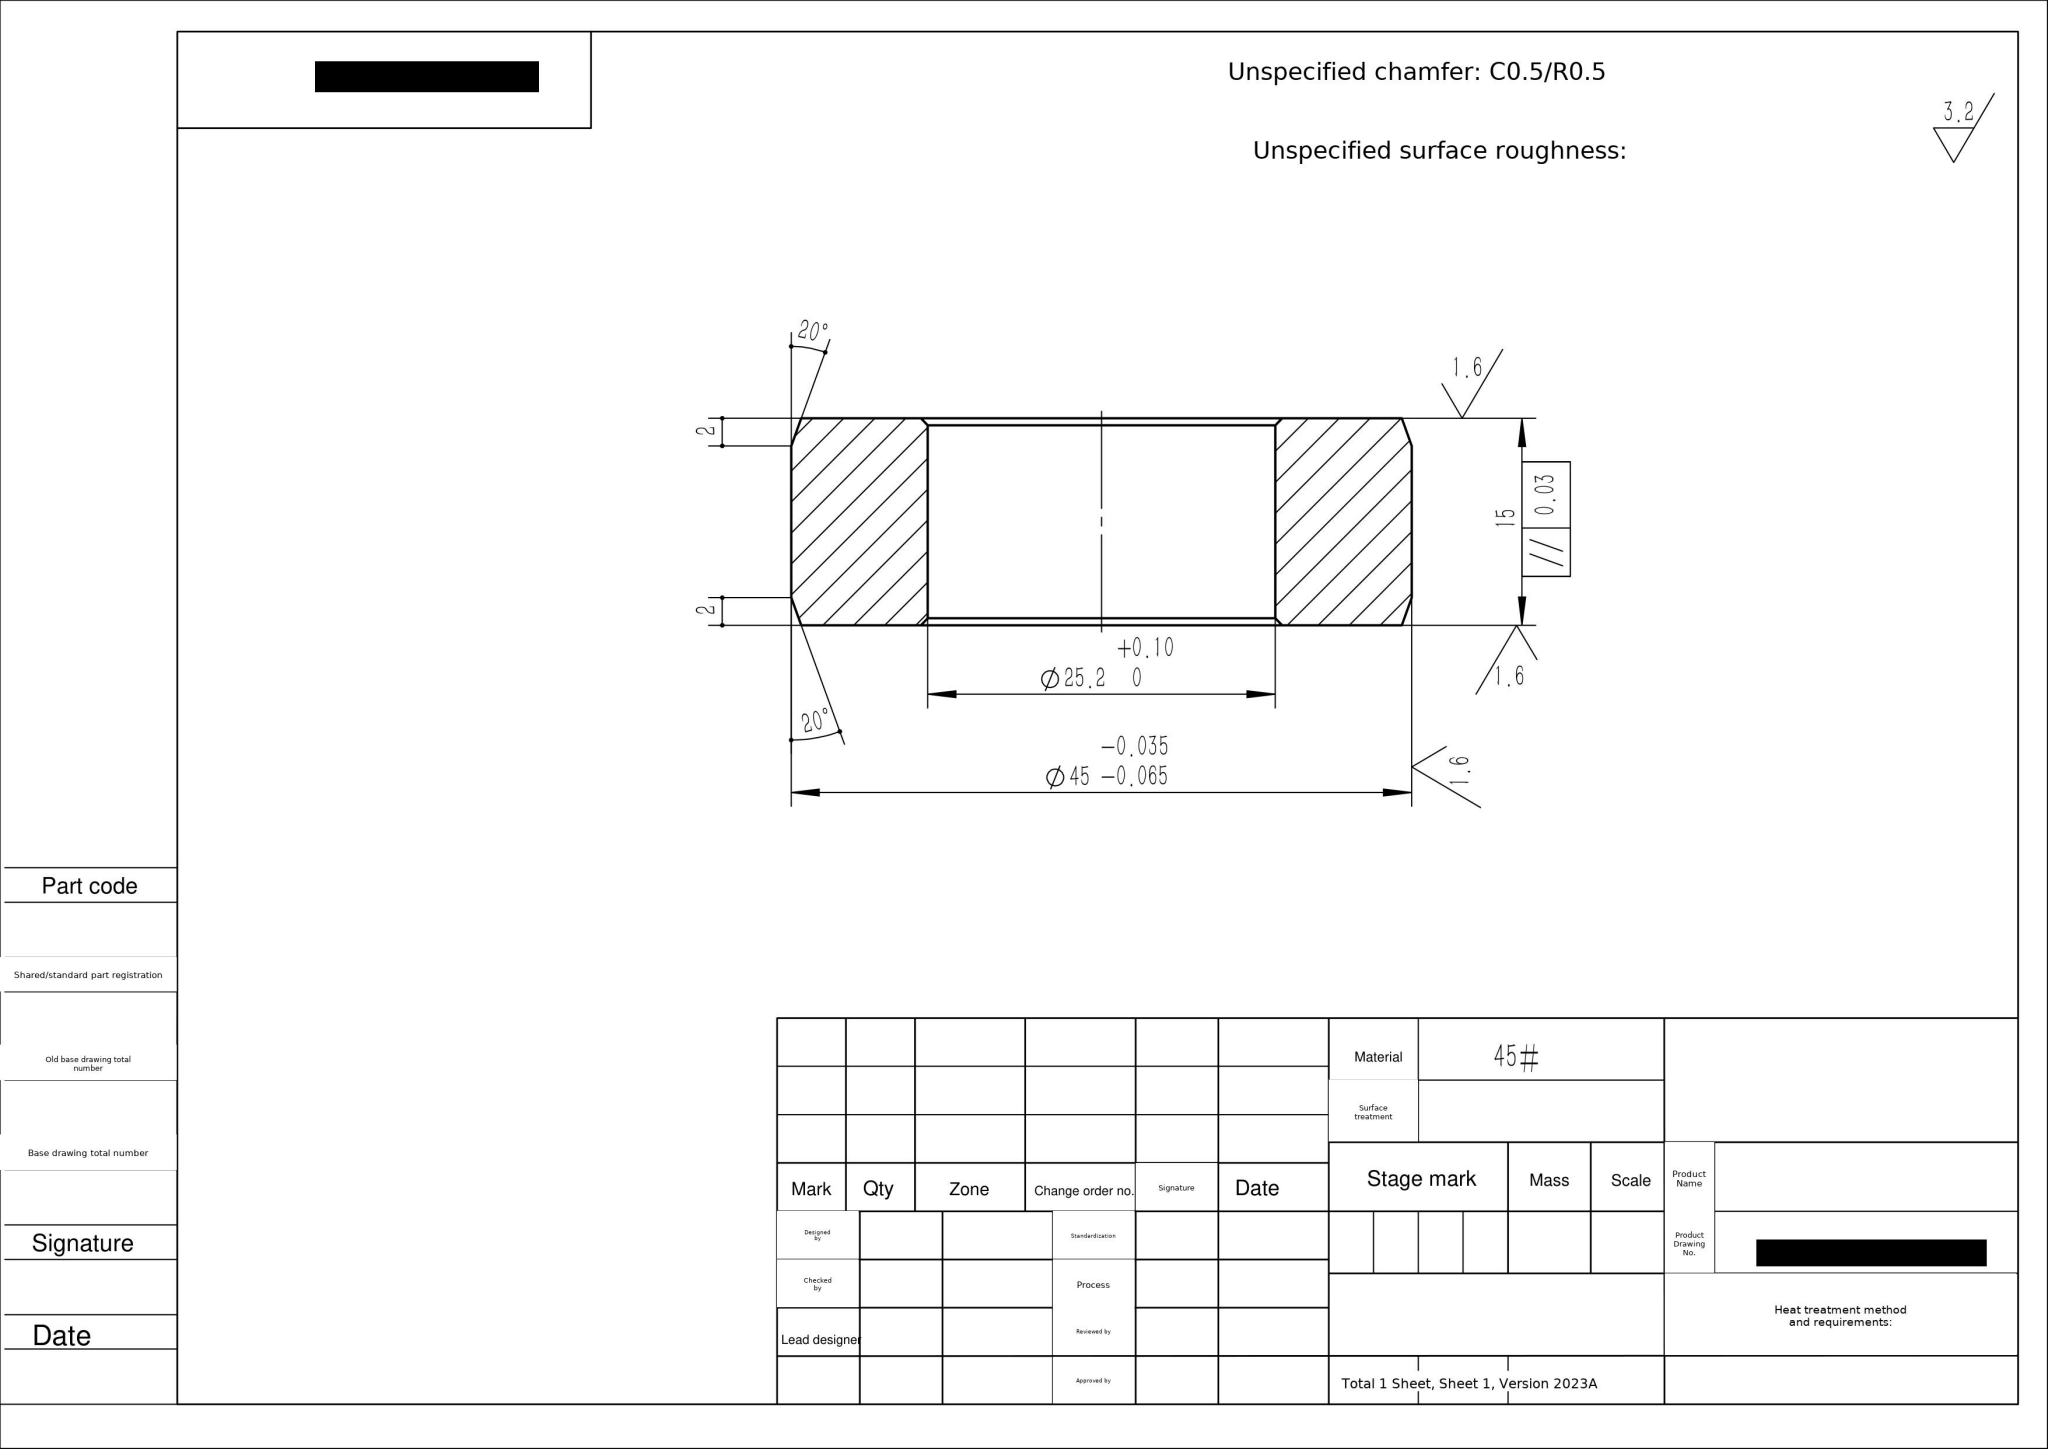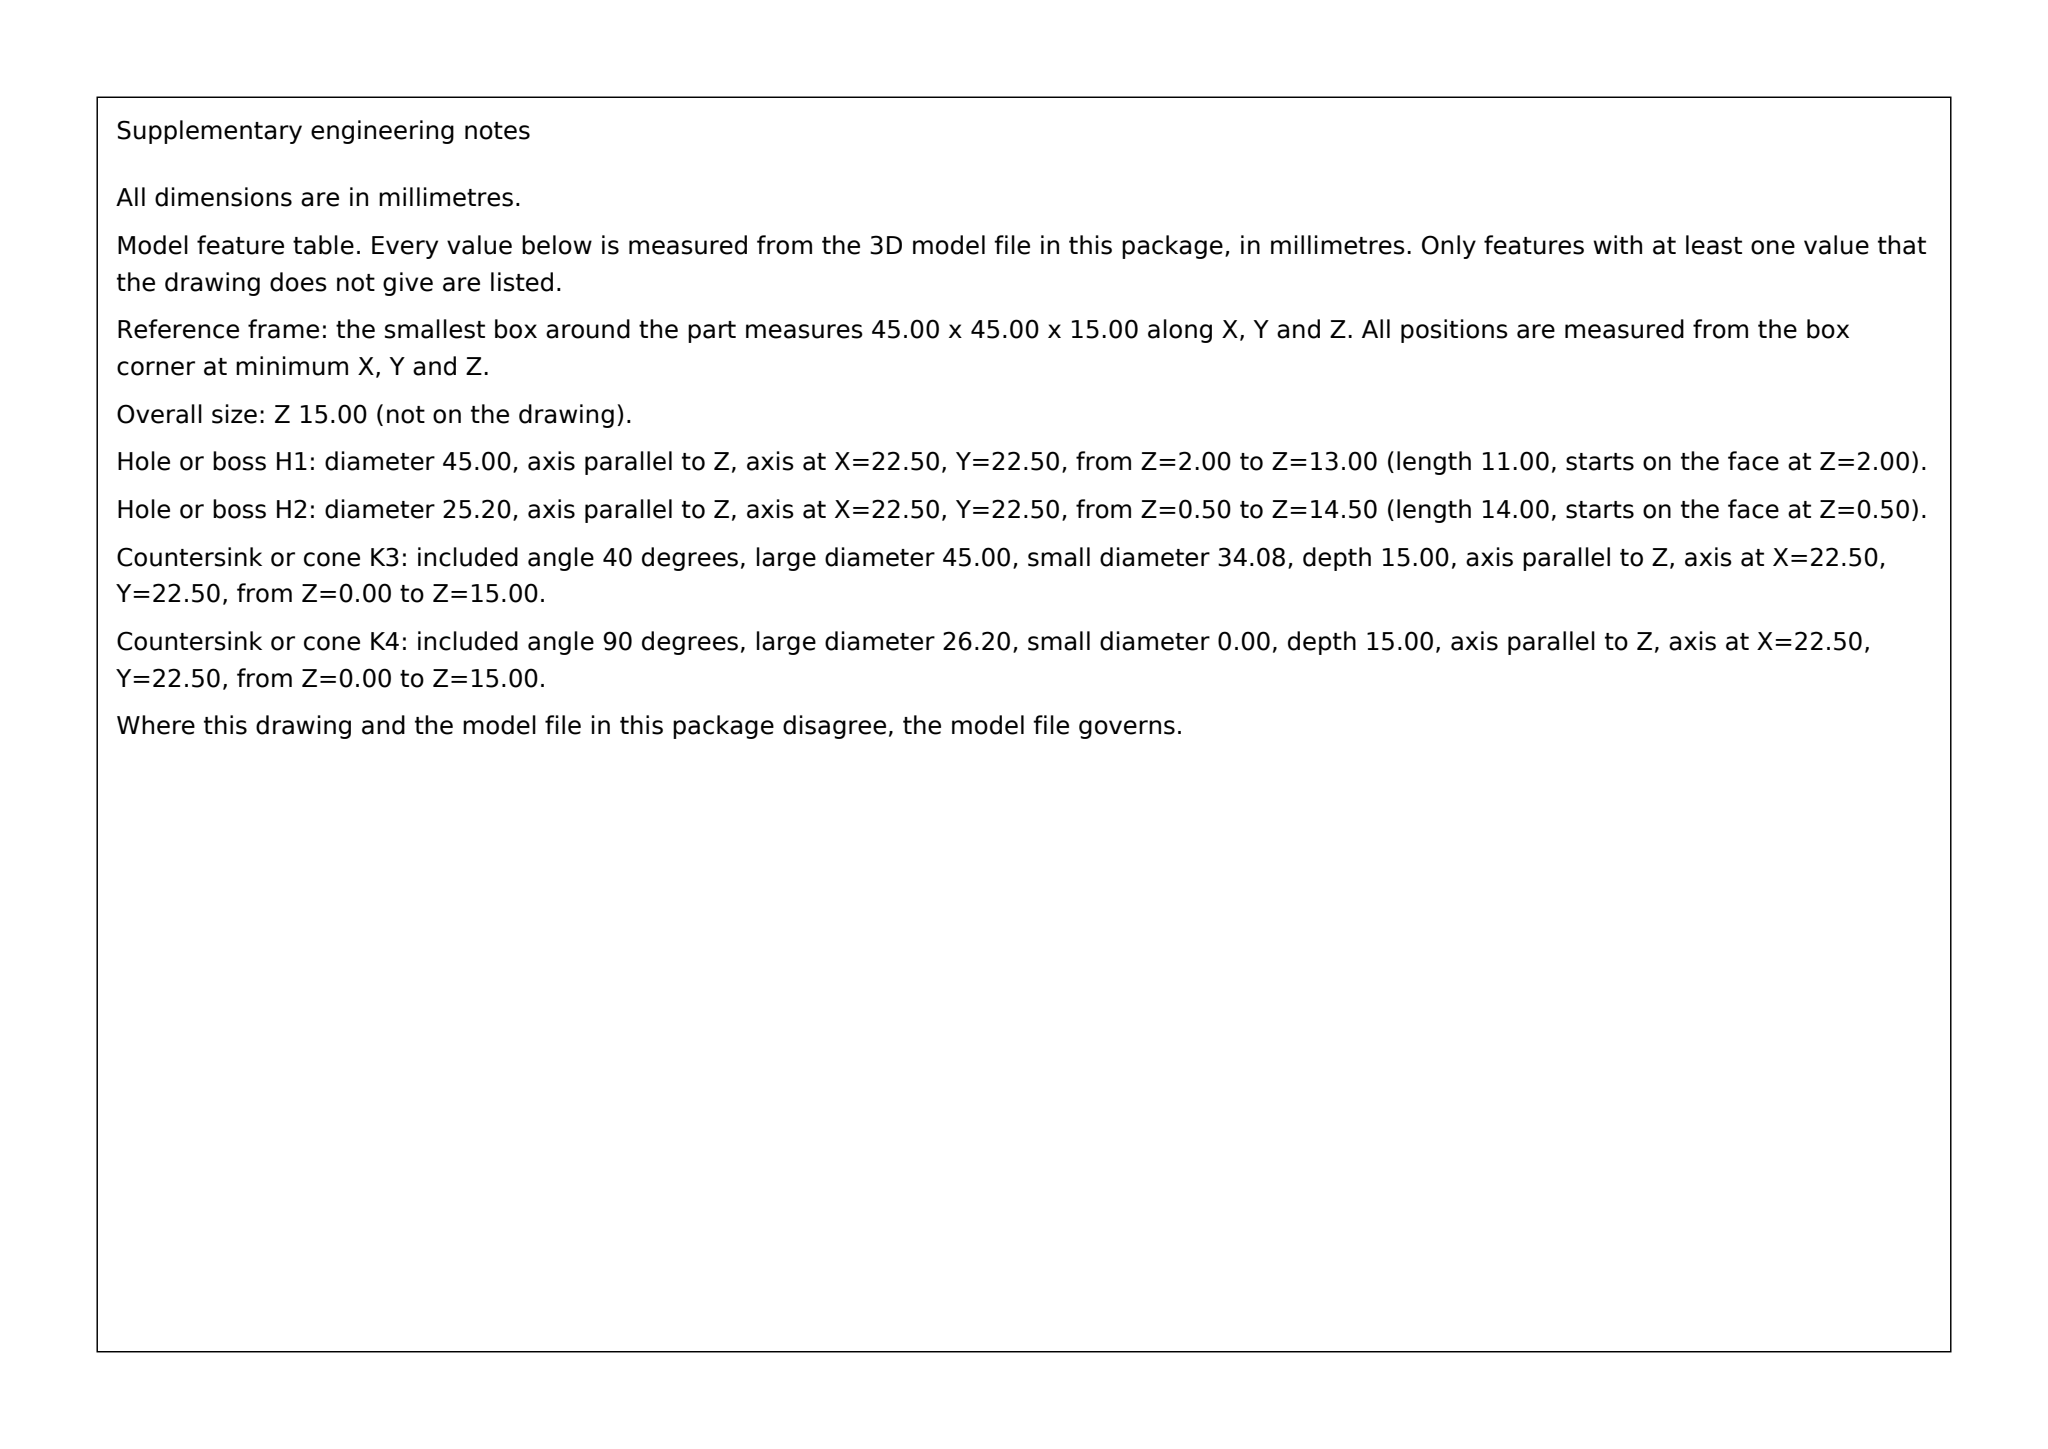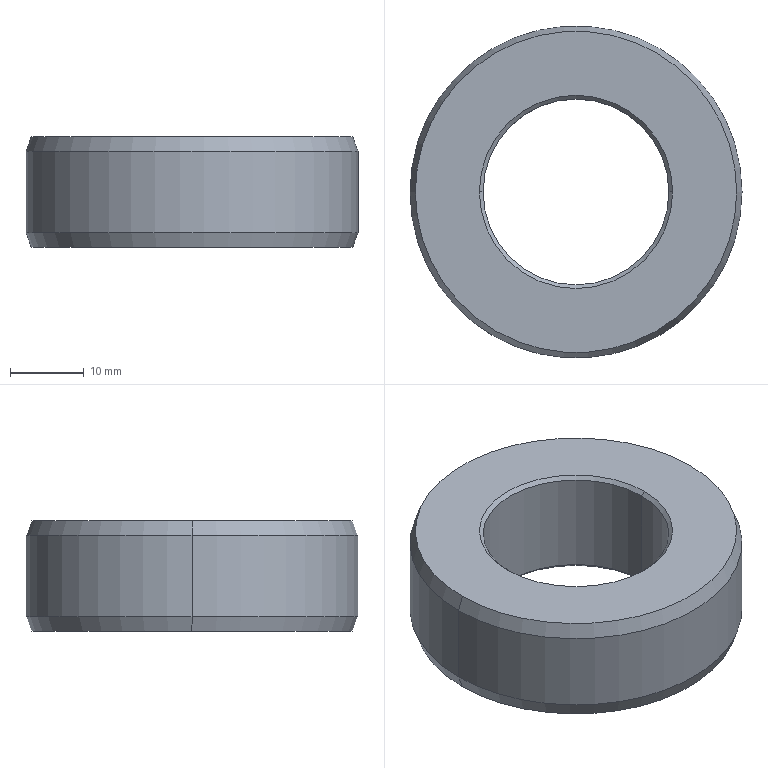Part | SolidWorks | mm | material 45# | 1 solid | 14 faces | box 45 x 45 x 15 mm | volume 16151 mm3 | cone 8 | cylinder 4 | plane 2 | commonest cylinder face diameters 25.2 x2 45 x2
build123d program:
from build123d import *

# Parameters (mm, degrees)
SKETCH1_R           = 22.5
SKETCH1_R_2         = 12.6
BOSS_EXTRUDE1_DEPTH = 15
CHAMFER1_SIZE       = 0.5
CHAMFER3_SIZE       = 2
CHAMFER3_SIZE2      = 0.7279
CHAMFER4_SIZE       = 2
CHAMFER4_SIZE2      = 0.7279


with BuildPart() as part:
    # Sketch1 → Boss-Extrude1 (new body)
    with BuildSketch(Plane.XY):
        Circle(SKETCH1_R)
        Circle(SKETCH1_R_2, mode=Mode.SUBTRACT)
    extrude(amount=BOSS_EXTRUDE1_DEPTH)

    # Chamfer1
    chamfer1_edges = [part.edges().sort_by_distance(p)[0] for p in [
        (-12.6, 0, 0),
        (-12.6, 0, 15),
    ]]
    chamfer(chamfer1_edges, length=CHAMFER1_SIZE)

    # Chamfer3
    chamfer3_edges = [part.edges().sort_by_distance(p)[0] for p in [
        (-22.5, 0, 15),
    ]]
    chamfer3_side = [part.faces().sort_by_distance(p)[0] for p in [
        (-22.5, 0, 7.5),
    ]]
    chamfer(chamfer3_edges, length=CHAMFER3_SIZE, length2=CHAMFER3_SIZE2, reference=chamfer3_side[0])

    # Chamfer4
    chamfer4_edges = [part.edges().sort_by_distance(p)[0] for p in [
        (-22.5, 0, 0),
    ]]
    chamfer4_side = [part.faces().sort_by_distance(p)[0] for p in [
        (-22.5, 0, 6.5),
    ]]
    chamfer(chamfer4_edges, length=CHAMFER4_SIZE, length2=CHAMFER4_SIZE2, reference=chamfer4_side[0])


solid = part.part
STEP:
#1=CARTESIAN_POINT('',(-21.772,0.,0.));
#2=VERTEX_POINT('',#1);
#3=CARTESIAN_POINT('',(21.772,0.,0.));
#4=VERTEX_POINT('',#3);
#5=CARTESIAN_POINT('',(0.,0.,0.));
#6=DIRECTION('',(0.,0.,-1.));
#7=DIRECTION('',(1.,0.,0.));
#8=AXIS2_PLACEMENT_3D('',#5,#6,#7);
#9=CIRCLE('',#8,21.772);
#10=EDGE_CURVE('',#2,#4,#9,.T.);
#11=ORIENTED_EDGE('',*,*,#10,.F.);
#12=CARTESIAN_POINT('',(-22.5,0.,2.));
#13=VERTEX_POINT('',#12);
#14=CARTESIAN_POINT('',(-22.5,0.,2.));
#15=DIRECTION('',(-0.342,0.,0.9397));
#16=VECTOR('',#15,1000.);
#17=LINE('',#14,#16);
#18=EDGE_CURVE('',#2,#13,#17,.T.);
#19=ORIENTED_EDGE('',*,*,#18,.T.);
#20=CARTESIAN_POINT('',(22.5,0.,2.));
#21=VERTEX_POINT('',#20);
#22=CARTESIAN_POINT('',(0.,0.,2.));
#23=DIRECTION('',(0.,0.,1.));
#24=DIRECTION('',(1.,0.,0.));
#25=AXIS2_PLACEMENT_3D('',#22,#23,#24);
#26=CIRCLE('',#25,22.5);
#27=EDGE_CURVE('',#21,#13,#26,.T.);
#28=ORIENTED_EDGE('',*,*,#27,.F.);
#29=CARTESIAN_POINT('',(22.5,0.,2.));
#30=DIRECTION('',(0.342,0.,0.9397));
#31=VECTOR('',#30,1000.);
#32=LINE('',#29,#31);
#33=EDGE_CURVE('',#4,#21,#32,.T.);
#34=ORIENTED_EDGE('',*,*,#33,.F.);
#35=EDGE_LOOP('',(#11,#19,#28,#34));
#36=FACE_OUTER_BOUND('',#35,.T.);
#37=CARTESIAN_POINT('',(0.,0.,2.));
#38=DIRECTION('',(0.,0.,1.));
#39=DIRECTION('',(1.,0.,0.));
#40=AXIS2_PLACEMENT_3D('',#37,#38,#39);
#41=CONICAL_SURFACE('',#40,22.5,0.3491);
#42=ADVANCED_FACE('',(#36),#41,.T.);
#43=CARTESIAN_POINT('',(21.772,0.,15.));
#44=VERTEX_POINT('',#43);
#45=CARTESIAN_POINT('',(-21.772,0.,15.));
#46=VERTEX_POINT('',#45);
#47=CARTESIAN_POINT('',(0.,0.,15.));
#48=DIRECTION('',(0.,0.,1.));
#49=DIRECTION('',(1.,0.,0.));
#50=AXIS2_PLACEMENT_3D('',#47,#48,#49);
#51=CIRCLE('',#50,21.772);
#52=EDGE_CURVE('',#44,#46,#51,.T.);
#53=ORIENTED_EDGE('',*,*,#52,.F.);
#54=CARTESIAN_POINT('',(22.5,0.,13.));
#55=VERTEX_POINT('',#54);
#56=CARTESIAN_POINT('',(21.772,0.,15.));
#57=DIRECTION('',(0.342,0.,-0.9397));
#58=VECTOR('',#57,1000.);
#59=LINE('',#56,#58);
#60=EDGE_CURVE('',#44,#55,#59,.T.);
#61=ORIENTED_EDGE('',*,*,#60,.T.);
#62=CARTESIAN_POINT('',(-22.5,0.,13.));
#63=VERTEX_POINT('',#62);
#64=CARTESIAN_POINT('',(0.,0.,13.));
#65=DIRECTION('',(0.,0.,-1.));
#66=DIRECTION('',(1.,0.,0.));
#67=AXIS2_PLACEMENT_3D('',#64,#65,#66);
#68=CIRCLE('',#67,22.5);
#69=EDGE_CURVE('',#63,#55,#68,.T.);
#70=ORIENTED_EDGE('',*,*,#69,.F.);
#71=CARTESIAN_POINT('',(-21.772,0.,15.));
#72=DIRECTION('',(-0.342,0.,-0.9397));
#73=VECTOR('',#72,1000.);
#74=LINE('',#71,#73);
#75=EDGE_CURVE('',#46,#63,#74,.T.);
#76=ORIENTED_EDGE('',*,*,#75,.F.);
#77=EDGE_LOOP('',(#53,#61,#70,#76));
#78=FACE_OUTER_BOUND('',#77,.T.);
#79=CARTESIAN_POINT('',(0.,0.,15.));
#80=DIRECTION('',(0.,0.,-1.));
#81=DIRECTION('',(-1.,0.,0.));
#82=AXIS2_PLACEMENT_3D('',#79,#80,#81);
#83=CONICAL_SURFACE('',#82,21.772,0.3491);
#84=ADVANCED_FACE('',(#78),#83,.T.);
#85=CARTESIAN_POINT('',(-12.6,0.,14.5));
#86=VERTEX_POINT('',#85);
#87=CARTESIAN_POINT('',(12.6,0.,14.5));
#88=VERTEX_POINT('',#87);
#89=CARTESIAN_POINT('',(0.,0.,14.5));
#90=DIRECTION('',(0.,0.,1.));
#91=DIRECTION('',(1.,0.,0.));
#92=AXIS2_PLACEMENT_3D('',#89,#90,#91);
#93=CIRCLE('',#92,12.6);
#94=EDGE_CURVE('',#86,#88,#93,.T.);
#95=ORIENTED_EDGE('',*,*,#94,.F.);
#96=CARTESIAN_POINT('',(-13.1,0.,15.));
#97=VERTEX_POINT('',#96);
#98=CARTESIAN_POINT('',(-12.6,0.,14.5));
#99=DIRECTION('',(-0.7071,0.,0.7071));
#100=VECTOR('',#99,1000.);
#101=LINE('',#98,#100);
#102=EDGE_CURVE('',#86,#97,#101,.T.);
#103=ORIENTED_EDGE('',*,*,#102,.T.);
#104=CARTESIAN_POINT('',(13.1,0.,15.));
#105=VERTEX_POINT('',#104);
#106=CARTESIAN_POINT('',(0.,0.,15.));
#107=DIRECTION('',(0.,0.,-1.));
#108=DIRECTION('',(1.,0.,0.));
#109=AXIS2_PLACEMENT_3D('',#106,#107,#108);
#110=CIRCLE('',#109,13.1);
#111=EDGE_CURVE('',#105,#97,#110,.T.);
#112=ORIENTED_EDGE('',*,*,#111,.F.);
#113=CARTESIAN_POINT('',(12.6,0.,14.5));
#114=DIRECTION('',(0.7071,0.,0.7071));
#115=VECTOR('',#114,1000.);
#116=LINE('',#113,#115);
#117=EDGE_CURVE('',#88,#105,#116,.T.);
#118=ORIENTED_EDGE('',*,*,#117,.F.);
#119=EDGE_LOOP('',(#95,#103,#112,#118));
#120=FACE_OUTER_BOUND('',#119,.T.);
#121=CARTESIAN_POINT('',(0.,0.,14.5));
#122=DIRECTION('',(0.,0.,1.));
#123=DIRECTION('',(1.,0.,0.));
#124=AXIS2_PLACEMENT_3D('',#121,#122,#123);
#125=CONICAL_SURFACE('',#124,12.6,0.7854);
#126=ADVANCED_FACE('',(#120),#125,.F.);
#127=CARTESIAN_POINT('',(12.6,0.,0.5));
#128=VERTEX_POINT('',#127);
#129=CARTESIAN_POINT('',(-12.6,0.,0.5));
#130=VERTEX_POINT('',#129);
#131=CARTESIAN_POINT('',(0.,0.,0.5));
#132=DIRECTION('',(0.,0.,-1.));
#133=DIRECTION('',(1.,0.,0.));
#134=AXIS2_PLACEMENT_3D('',#131,#132,#133);
#135=CIRCLE('',#134,12.6);
#136=EDGE_CURVE('',#128,#130,#135,.T.);
#137=ORIENTED_EDGE('',*,*,#136,.F.);
#138=CARTESIAN_POINT('',(13.1,0.,0.));
#139=VERTEX_POINT('',#138);
#140=CARTESIAN_POINT('',(13.1,0.,0.));
#141=DIRECTION('',(0.7071,0.,-0.7071));
#142=VECTOR('',#141,1000.);
#143=LINE('',#140,#142);
#144=EDGE_CURVE('',#128,#139,#143,.T.);
#145=ORIENTED_EDGE('',*,*,#144,.T.);
#146=CARTESIAN_POINT('',(-13.1,0.,0.));
#147=VERTEX_POINT('',#146);
#148=CARTESIAN_POINT('',(0.,0.,0.));
#149=DIRECTION('',(0.,0.,1.));
#150=DIRECTION('',(1.,0.,0.));
#151=AXIS2_PLACEMENT_3D('',#148,#149,#150);
#152=CIRCLE('',#151,13.1);
#153=EDGE_CURVE('',#147,#139,#152,.T.);
#154=ORIENTED_EDGE('',*,*,#153,.F.);
#155=CARTESIAN_POINT('',(-13.1,0.,0.));
#156=DIRECTION('',(-0.7071,0.,-0.7071));
#157=VECTOR('',#156,1000.);
#158=LINE('',#155,#157);
#159=EDGE_CURVE('',#130,#147,#158,.T.);
#160=ORIENTED_EDGE('',*,*,#159,.F.);
#161=EDGE_LOOP('',(#137,#145,#154,#160));
#162=FACE_OUTER_BOUND('',#161,.T.);
#163=CARTESIAN_POINT('',(0.,0.,0.));
#164=DIRECTION('',(0.,0.,-1.));
#165=DIRECTION('',(-1.,0.,0.));
#166=AXIS2_PLACEMENT_3D('',#163,#164,#165);
#167=CONICAL_SURFACE('',#166,13.1,0.7854);
#168=ADVANCED_FACE('',(#162),#167,.F.);
#169=ORIENTED_EDGE('',*,*,#94,.T.);
#170=CARTESIAN_POINT('',(12.6,0.,15.));
#171=DIRECTION('',(0.,0.,-1.));
#172=VECTOR('',#171,1000.);
#173=LINE('',#170,#172);
#174=EDGE_CURVE('',#88,#128,#173,.T.);
#175=ORIENTED_EDGE('',*,*,#174,.T.);
#176=ORIENTED_EDGE('',*,*,#136,.T.);
#177=CARTESIAN_POINT('',(-12.6,0.,15.));
#178=DIRECTION('',(0.,0.,-1.));
#179=VECTOR('',#178,1000.);
#180=LINE('',#177,#179);
#181=EDGE_CURVE('',#86,#130,#180,.T.);
#182=ORIENTED_EDGE('',*,*,#181,.F.);
#183=EDGE_LOOP('',(#169,#175,#176,#182));
#184=FACE_OUTER_BOUND('',#183,.T.);
#185=CARTESIAN_POINT('',(0.,0.,15.));
#186=DIRECTION('',(0.,0.,-1.));
#187=DIRECTION('',(-1.,0.,0.));
#188=AXIS2_PLACEMENT_3D('',#185,#186,#187);
#189=CYLINDRICAL_SURFACE('',#188,12.6);
#190=ADVANCED_FACE('',(#184),#189,.F.);
#191=ORIENTED_EDGE('',*,*,#69,.T.);
#192=CARTESIAN_POINT('',(22.5,0.,15.));
#193=DIRECTION('',(0.,0.,-1.));
#194=VECTOR('',#193,1000.);
#195=LINE('',#192,#194);
#196=EDGE_CURVE('',#55,#21,#195,.T.);
#197=ORIENTED_EDGE('',*,*,#196,.T.);
#198=ORIENTED_EDGE('',*,*,#27,.T.);
#199=CARTESIAN_POINT('',(-22.5,0.,15.));
#200=DIRECTION('',(0.,0.,-1.));
#201=VECTOR('',#200,1000.);
#202=LINE('',#199,#201);
#203=EDGE_CURVE('',#63,#13,#202,.T.);
#204=ORIENTED_EDGE('',*,*,#203,.F.);
#205=EDGE_LOOP('',(#191,#197,#198,#204));
#206=FACE_OUTER_BOUND('',#205,.T.);
#207=CARTESIAN_POINT('',(0.,0.,15.));
#208=DIRECTION('',(0.,0.,-1.));
#209=DIRECTION('',(-1.,0.,0.));
#210=AXIS2_PLACEMENT_3D('',#207,#208,#209);
#211=CYLINDRICAL_SURFACE('',#210,22.5);
#212=ADVANCED_FACE('',(#206),#211,.T.);
#213=CARTESIAN_POINT('',(0.,0.,15.));
#214=DIRECTION('',(0.,0.,1.));
#215=DIRECTION('',(1.,0.,0.));
#216=AXIS2_PLACEMENT_3D('',#213,#214,#215);
#217=CIRCLE('',#216,21.772);
#218=EDGE_CURVE('',#46,#44,#217,.T.);
#219=ORIENTED_EDGE('',*,*,#218,.T.);
#220=ORIENTED_EDGE('',*,*,#52,.T.);
#221=EDGE_LOOP('',(#219,#220));
#222=FACE_OUTER_BOUND('',#221,.T.);
#223=ORIENTED_EDGE('',*,*,#111,.T.);
#224=CARTESIAN_POINT('',(0.,0.,15.));
#225=DIRECTION('',(0.,0.,-1.));
#226=DIRECTION('',(1.,0.,0.));
#227=AXIS2_PLACEMENT_3D('',#224,#225,#226);
#228=CIRCLE('',#227,13.1);
#229=EDGE_CURVE('',#97,#105,#228,.T.);
#230=ORIENTED_EDGE('',*,*,#229,.T.);
#231=EDGE_LOOP('',(#223,#230));
#232=FACE_BOUND('',#231,.T.);
#233=CARTESIAN_POINT('',(0.,0.,15.));
#234=DIRECTION('',(0.,0.,1.));
#235=DIRECTION('',(1.,0.,0.));
#236=AXIS2_PLACEMENT_3D('',#233,#234,#235);
#237=PLANE('',#236);
#238=ADVANCED_FACE('',(#222,#232),#237,.T.);
#239=CARTESIAN_POINT('',(0.,0.,0.));
#240=DIRECTION('',(0.,0.,-1.));
#241=DIRECTION('',(1.,0.,0.));
#242=AXIS2_PLACEMENT_3D('',#239,#240,#241);
#243=CIRCLE('',#242,21.772);
#244=EDGE_CURVE('',#4,#2,#243,.T.);
#245=ORIENTED_EDGE('',*,*,#244,.T.);
#246=ORIENTED_EDGE('',*,*,#10,.T.);
#247=EDGE_LOOP('',(#245,#246));
#248=FACE_OUTER_BOUND('',#247,.T.);
#249=ORIENTED_EDGE('',*,*,#153,.T.);
#250=CARTESIAN_POINT('',(0.,0.,0.));
#251=DIRECTION('',(0.,0.,1.));
#252=DIRECTION('',(1.,0.,0.));
#253=AXIS2_PLACEMENT_3D('',#250,#251,#252);
#254=CIRCLE('',#253,13.1);
#255=EDGE_CURVE('',#139,#147,#254,.T.);
#256=ORIENTED_EDGE('',*,*,#255,.T.);
#257=EDGE_LOOP('',(#249,#256));
#258=FACE_BOUND('',#257,.T.);
#259=CARTESIAN_POINT('',(0.,0.,0.));
#260=DIRECTION('',(0.,0.,1.));
#261=DIRECTION('',(1.,0.,0.));
#262=AXIS2_PLACEMENT_3D('',#259,#260,#261);
#263=PLANE('',#262);
#264=ADVANCED_FACE('',(#248,#258),#263,.F.);
#265=ORIENTED_EDGE('',*,*,#196,.F.);
#266=CARTESIAN_POINT('',(0.,0.,13.));
#267=DIRECTION('',(0.,0.,-1.));
#268=DIRECTION('',(1.,0.,0.));
#269=AXIS2_PLACEMENT_3D('',#266,#267,#268);
#270=CIRCLE('',#269,22.5);
#271=EDGE_CURVE('',#55,#63,#270,.T.);
#272=ORIENTED_EDGE('',*,*,#271,.T.);
#273=ORIENTED_EDGE('',*,*,#203,.T.);
#274=CARTESIAN_POINT('',(0.,0.,2.));
#275=DIRECTION('',(0.,0.,1.));
#276=DIRECTION('',(1.,0.,0.));
#277=AXIS2_PLACEMENT_3D('',#274,#275,#276);
#278=CIRCLE('',#277,22.5);
#279=EDGE_CURVE('',#13,#21,#278,.T.);
#280=ORIENTED_EDGE('',*,*,#279,.T.);
#281=EDGE_LOOP('',(#265,#272,#273,#280));
#282=FACE_OUTER_BOUND('',#281,.T.);
#283=CARTESIAN_POINT('',(0.,0.,15.));
#284=DIRECTION('',(0.,0.,-1.));
#285=DIRECTION('',(-1.,0.,0.));
#286=AXIS2_PLACEMENT_3D('',#283,#284,#285);
#287=CYLINDRICAL_SURFACE('',#286,22.5);
#288=ADVANCED_FACE('',(#282),#287,.T.);
#289=ORIENTED_EDGE('',*,*,#174,.F.);
#290=CARTESIAN_POINT('',(0.,0.,14.5));
#291=DIRECTION('',(0.,0.,1.));
#292=DIRECTION('',(1.,0.,0.));
#293=AXIS2_PLACEMENT_3D('',#290,#291,#292);
#294=CIRCLE('',#293,12.6);
#295=EDGE_CURVE('',#88,#86,#294,.T.);
#296=ORIENTED_EDGE('',*,*,#295,.T.);
#297=ORIENTED_EDGE('',*,*,#181,.T.);
#298=CARTESIAN_POINT('',(0.,0.,0.5));
#299=DIRECTION('',(0.,0.,-1.));
#300=DIRECTION('',(1.,0.,0.));
#301=AXIS2_PLACEMENT_3D('',#298,#299,#300);
#302=CIRCLE('',#301,12.6);
#303=EDGE_CURVE('',#130,#128,#302,.T.);
#304=ORIENTED_EDGE('',*,*,#303,.T.);
#305=EDGE_LOOP('',(#289,#296,#297,#304));
#306=FACE_OUTER_BOUND('',#305,.T.);
#307=CARTESIAN_POINT('',(0.,0.,15.));
#308=DIRECTION('',(0.,0.,-1.));
#309=DIRECTION('',(-1.,0.,0.));
#310=AXIS2_PLACEMENT_3D('',#307,#308,#309);
#311=CYLINDRICAL_SURFACE('',#310,12.6);
#312=ADVANCED_FACE('',(#306),#311,.F.);
#313=ORIENTED_EDGE('',*,*,#144,.F.);
#314=ORIENTED_EDGE('',*,*,#303,.F.);
#315=ORIENTED_EDGE('',*,*,#159,.T.);
#316=ORIENTED_EDGE('',*,*,#255,.F.);
#317=EDGE_LOOP('',(#313,#314,#315,#316));
#318=FACE_OUTER_BOUND('',#317,.T.);
#319=CARTESIAN_POINT('',(0.,0.,0.));
#320=DIRECTION('',(0.,0.,-1.));
#321=DIRECTION('',(-1.,0.,0.));
#322=AXIS2_PLACEMENT_3D('',#319,#320,#321);
#323=CONICAL_SURFACE('',#322,13.1,0.7854);
#324=ADVANCED_FACE('',(#318),#323,.F.);
#325=ORIENTED_EDGE('',*,*,#102,.F.);
#326=ORIENTED_EDGE('',*,*,#295,.F.);
#327=ORIENTED_EDGE('',*,*,#117,.T.);
#328=ORIENTED_EDGE('',*,*,#229,.F.);
#329=EDGE_LOOP('',(#325,#326,#327,#328));
#330=FACE_OUTER_BOUND('',#329,.T.);
#331=CARTESIAN_POINT('',(0.,0.,14.5));
#332=DIRECTION('',(0.,0.,1.));
#333=DIRECTION('',(1.,0.,0.));
#334=AXIS2_PLACEMENT_3D('',#331,#332,#333);
#335=CONICAL_SURFACE('',#334,12.6,0.7854);
#336=ADVANCED_FACE('',(#330),#335,.F.);
#337=ORIENTED_EDGE('',*,*,#60,.F.);
#338=ORIENTED_EDGE('',*,*,#218,.F.);
#339=ORIENTED_EDGE('',*,*,#75,.T.);
#340=ORIENTED_EDGE('',*,*,#271,.F.);
#341=EDGE_LOOP('',(#337,#338,#339,#340));
#342=FACE_OUTER_BOUND('',#341,.T.);
#343=CARTESIAN_POINT('',(0.,0.,15.));
#344=DIRECTION('',(0.,0.,-1.));
#345=DIRECTION('',(-1.,0.,0.));
#346=AXIS2_PLACEMENT_3D('',#343,#344,#345);
#347=CONICAL_SURFACE('',#346,21.772,0.3491);
#348=ADVANCED_FACE('',(#342),#347,.T.);
#349=ORIENTED_EDGE('',*,*,#18,.F.);
#350=ORIENTED_EDGE('',*,*,#244,.F.);
#351=ORIENTED_EDGE('',*,*,#33,.T.);
#352=ORIENTED_EDGE('',*,*,#279,.F.);
#353=EDGE_LOOP('',(#349,#350,#351,#352));
#354=FACE_OUTER_BOUND('',#353,.T.);
#355=CARTESIAN_POINT('',(0.,0.,2.));
#356=DIRECTION('',(0.,0.,1.));
#357=DIRECTION('',(1.,0.,0.));
#358=AXIS2_PLACEMENT_3D('',#355,#356,#357);
#359=CONICAL_SURFACE('',#358,22.5,0.3491);
#360=ADVANCED_FACE('',(#354),#359,.T.);
#361=CLOSED_SHELL('',(#42,#84,#126,#168,#190,#212,#238,#264,#288,#312,#324,#336,#348,#360));
#362=MANIFOLD_SOLID_BREP('',#361);
#363=CARTESIAN_POINT('',(0.,0.,0.));
#364=DIRECTION('',(0.,0.,1.));
#365=DIRECTION('',(1.,0.,0.));
#366=AXIS2_PLACEMENT_3D('',#363,#364,#365);
#367=(LENGTH_UNIT()NAMED_UNIT(*)SI_UNIT(.MILLI.,.METRE.));
#368=UNCERTAINTY_MEASURE_WITH_UNIT(LENGTH_MEASURE(0.00001),#367,'','');
#369=(NAMED_UNIT(*)PLANE_ANGLE_UNIT()SI_UNIT($,.RADIAN.));
#370=(NAMED_UNIT(*)SI_UNIT($,.STERADIAN.)SOLID_ANGLE_UNIT());
#371=(GEOMETRIC_REPRESENTATION_CONTEXT(3)GLOBAL_UNCERTAINTY_ASSIGNED_CONTEXT((#368))GLOBAL_UNIT_ASSIGNED_CONTEXT((#367,#369,#370))REPRESENTATION_CONTEXT('',''));
#372=ADVANCED_BREP_SHAPE_REPRESENTATION('',(#362,#366),#371);